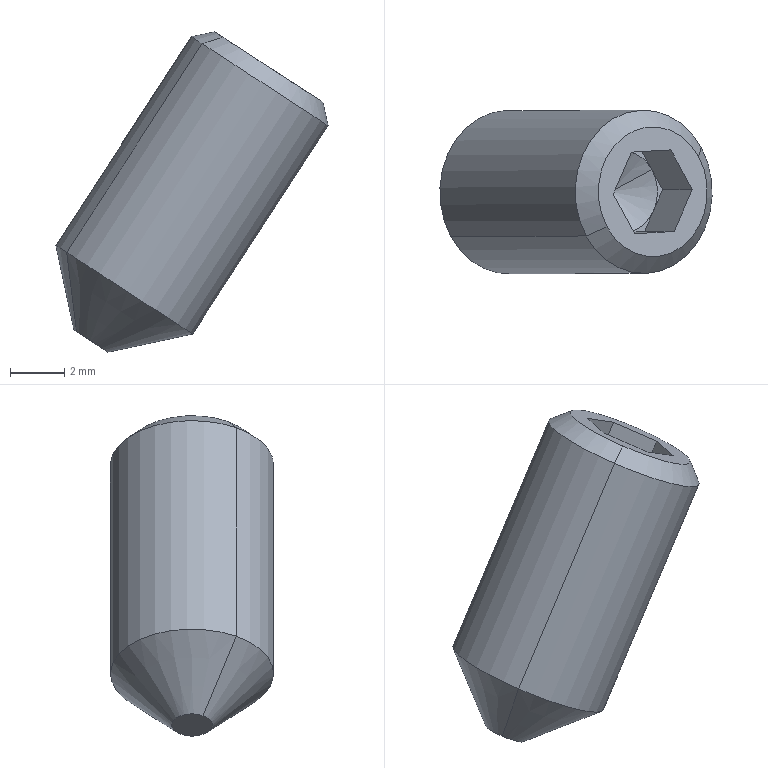Component | SolidWorks | SetScrewTAY12-M6-L12(YIHEDA)-1 | 1 solid | 22 faces | box 10.01 x 6 x 11.77 mm | volume 283 mm3 | plane 14 | cone 6 | cylinder 2 | commonest cylinder face diameters 6 x2
STEP:
#1=CARTESIAN_POINT('',(4.498,-0.6106,10.849));
#2=VERTEX_POINT('',#1);
#3=CARTESIAN_POINT('',(4.332,-0.7385,10.958));
#4=VERTEX_POINT('',#3);
#5=CARTESIAN_POINT('',(4.415,-0.6746,10.903));
#6=DIRECTION('',(-0.5446,0.,-0.8387));
#7=DIRECTION('',(-0.705,-0.5417,0.4578));
#8=AXIS2_PLACEMENT_3D('',#5,#6,#7);
#9=CIRCLE('',#8,0.1181);
#10=EDGE_CURVE('',#2,#4,#9,.T.);
#11=ORIENTED_EDGE('',*,*,#10,.F.);
#12=CARTESIAN_POINT('',(4.694,-0.6106,11.151));
#13=VERTEX_POINT('',#12);
#14=CARTESIAN_POINT('',(4.45,-0.6106,10.775));
#15=DIRECTION('',(0.5446,-0.,0.8387));
#16=VECTOR('',#15,39.37);
#17=LINE('',#14,#16);
#18=EDGE_CURVE('',#2,#13,#17,.T.);
#19=ORIENTED_EDGE('',*,*,#18,.T.);
#20=CARTESIAN_POINT('',(4.528,-0.7385,11.259));
#21=VERTEX_POINT('',#20);
#22=CARTESIAN_POINT('',(4.611,-0.6746,11.205));
#23=DIRECTION('',(-0.5446,0.,-0.8387));
#24=DIRECTION('',(-0.705,-0.5417,0.4578));
#25=AXIS2_PLACEMENT_3D('',#22,#23,#24);
#26=CIRCLE('',#25,0.1181);
#27=EDGE_CURVE('',#13,#21,#26,.T.);
#28=ORIENTED_EDGE('',*,*,#27,.T.);
#29=CARTESIAN_POINT('',(4.284,-0.7385,10.883));
#30=DIRECTION('',(0.5446,-0.,0.8387));
#31=VECTOR('',#30,39.37);
#32=LINE('',#29,#31);
#33=EDGE_CURVE('',#4,#21,#32,.T.);
#34=ORIENTED_EDGE('',*,*,#33,.F.);
#35=EDGE_LOOP('',(#11,#19,#28,#34));
#36=FACE_OUTER_BOUND('',#35,.T.);
#37=CARTESIAN_POINT('',(4.367,-0.6746,10.829));
#38=DIRECTION('',(0.5446,-0.,0.8387));
#39=DIRECTION('',(-0.705,-0.5417,0.4578));
#40=AXIS2_PLACEMENT_3D('',#37,#38,#39);
#41=CYLINDRICAL_SURFACE('',#40,0.1181);
#42=ADVANCED_FACE('',(#36),#41,.T.);
#43=CARTESIAN_POINT('',(4.346,-0.6906,10.843));
#44=VERTEX_POINT('',#43);
#45=CARTESIAN_POINT('',(4.388,-0.6586,10.816));
#46=VERTEX_POINT('',#45);
#47=CARTESIAN_POINT('',(4.367,-0.6746,10.829));
#48=DIRECTION('',(-0.5446,0.,-0.8387));
#49=DIRECTION('',(-0.705,-0.5417,0.4578));
#50=AXIS2_PLACEMENT_3D('',#47,#48,#49);
#51=CIRCLE('',#50,0.02953);
#52=EDGE_CURVE('',#44,#46,#51,.T.);
#53=ORIENTED_EDGE('',*,*,#52,.F.);
#54=CARTESIAN_POINT('',(4.332,-0.7385,10.958));
#55=DIRECTION('',(-0.1134,-0.3831,0.9167));
#56=VECTOR('',#55,39.37);
#57=LINE('',#54,#56);
#58=EDGE_CURVE('',#44,#4,#57,.T.);
#59=ORIENTED_EDGE('',*,*,#58,.T.);
#60=CARTESIAN_POINT('',(4.415,-0.6746,10.903));
#61=DIRECTION('',(-0.5446,0.,-0.8387));
#62=DIRECTION('',(-0.705,-0.5417,0.4578));
#63=AXIS2_PLACEMENT_3D('',#60,#61,#62);
#64=CIRCLE('',#63,0.1181);
#65=EDGE_CURVE('',#4,#2,#64,.T.);
#66=ORIENTED_EDGE('',*,*,#65,.T.);
#67=CARTESIAN_POINT('',(4.498,-0.6106,10.849));
#68=DIRECTION('',(0.8836,0.3831,0.2693));
#69=VECTOR('',#68,39.37);
#70=LINE('',#67,#69);
#71=EDGE_CURVE('',#46,#2,#70,.T.);
#72=ORIENTED_EDGE('',*,*,#71,.F.);
#73=EDGE_LOOP('',(#53,#59,#66,#72));
#74=FACE_OUTER_BOUND('',#73,.T.);
#75=CARTESIAN_POINT('',(4.415,-0.6746,10.903));
#76=DIRECTION('',(0.5446,-0.,0.8387));
#77=DIRECTION('',(0.705,0.5417,-0.4578));
#78=AXIS2_PLACEMENT_3D('',#75,#76,#77);
#79=CONICAL_SURFACE('',#78,0.1181,0.7854);
#80=ADVANCED_FACE('',(#74),#79,.T.);
#81=CARTESIAN_POINT('',(4.558,-0.7255,11.268));
#82=VERTEX_POINT('',#81);
#83=CARTESIAN_POINT('',(4.691,-0.6237,11.182));
#84=VERTEX_POINT('',#83);
#85=CARTESIAN_POINT('',(4.624,-0.6746,11.225));
#86=DIRECTION('',(-0.5446,0.,-0.8387));
#87=DIRECTION('',(-0.705,-0.5417,0.4578));
#88=AXIS2_PLACEMENT_3D('',#85,#86,#87);
#89=CIRCLE('',#88,0.09396);
#90=EDGE_CURVE('',#82,#84,#89,.T.);
#91=ORIENTED_EDGE('',*,*,#90,.T.);
#92=CARTESIAN_POINT('',(4.691,-0.6237,11.182));
#93=DIRECTION('',(0.1134,0.3831,-0.9167));
#94=VECTOR('',#93,39.37);
#95=LINE('',#92,#94);
#96=EDGE_CURVE('',#84,#13,#95,.T.);
#97=ORIENTED_EDGE('',*,*,#96,.T.);
#98=CARTESIAN_POINT('',(4.611,-0.6746,11.205));
#99=DIRECTION('',(-0.5446,0.,-0.8387));
#100=DIRECTION('',(-0.705,-0.5417,0.4578));
#101=AXIS2_PLACEMENT_3D('',#98,#99,#100);
#102=CIRCLE('',#101,0.1181);
#103=EDGE_CURVE('',#21,#13,#102,.T.);
#104=ORIENTED_EDGE('',*,*,#103,.F.);
#105=CARTESIAN_POINT('',(4.558,-0.7255,11.268));
#106=DIRECTION('',(-0.8836,-0.3831,-0.2693));
#107=VECTOR('',#106,39.37);
#108=LINE('',#105,#107);
#109=EDGE_CURVE('',#82,#21,#108,.T.);
#110=ORIENTED_EDGE('',*,*,#109,.F.);
#111=EDGE_LOOP('',(#91,#97,#104,#110));
#112=FACE_OUTER_BOUND('',#111,.T.);
#113=CARTESIAN_POINT('',(4.624,-0.6746,11.225));
#114=DIRECTION('',(-0.5446,0.,-0.8387));
#115=DIRECTION('',(-0.705,-0.5417,0.4578));
#116=AXIS2_PLACEMENT_3D('',#113,#114,#115);
#117=CONICAL_SURFACE('',#116,0.09396,0.7854);
#118=ADVANCED_FACE('',(#112),#117,.T.);
#119=CARTESIAN_POINT('',(4.563,-0.6746,11.131));
#120=VERTEX_POINT('',#119);
#121=CARTESIAN_POINT('',(4.623,-0.6426,11.132));
#122=VERTEX_POINT('',#121);
#123=CARTESIAN_POINT('',(4.623,-0.6426,11.132));
#124=DIRECTION('',(0.8818,0.4713,0.01518));
#125=VECTOR('',#124,39.37);
#126=LINE('',#123,#125);
#127=EDGE_CURVE('',#120,#122,#126,.T.);
#128=ORIENTED_EDGE('',*,*,#127,.F.);
#129=CARTESIAN_POINT('',(4.54,-0.7066,11.186));
#130=VERTEX_POINT('',#129);
#131=CARTESIAN_POINT('',(4.54,-0.7066,11.186));
#132=DIRECTION('',(-0.3448,-0.4713,0.8118));
#133=VECTOR('',#132,39.37);
#134=LINE('',#131,#133);
#135=EDGE_CURVE('',#120,#130,#134,.T.);
#136=ORIENTED_EDGE('',*,*,#135,.T.);
#137=CARTESIAN_POINT('',(4.584,-0.7336,11.158));
#138=VERTEX_POINT('',#137);
#139=CARTESIAN_POINT('',(4.581,-0.6746,11.159));
#140=DIRECTION('',(0.5446,-0.,0.8387));
#141=DIRECTION('',(-0.705,-0.5417,0.4578));
#142=AXIS2_PLACEMENT_3D('',#139,#140,#141);
#143=CIRCLE('',#142,0.05906);
#144=EDGE_CURVE('',#130,#138,#143,.T.);
#145=ORIENTED_EDGE('',*,*,#144,.T.);
#146=CARTESIAN_POINT('',(4.625,-0.7016,11.131));
#147=VERTEX_POINT('',#146);
#148=CARTESIAN_POINT('',(4.581,-0.6746,11.159));
#149=DIRECTION('',(0.5446,-0.,0.8387));
#150=DIRECTION('',(-0.705,-0.5417,0.4578));
#151=AXIS2_PLACEMENT_3D('',#148,#149,#150);
#152=CIRCLE('',#151,0.05906);
#153=EDGE_CURVE('',#138,#147,#152,.T.);
#154=ORIENTED_EDGE('',*,*,#153,.T.);
#155=CARTESIAN_POINT('',(4.581,-0.6746,11.159));
#156=DIRECTION('',(0.5446,-0.,0.8387));
#157=DIRECTION('',(-0.705,-0.5417,0.4578));
#158=AXIS2_PLACEMENT_3D('',#155,#156,#157);
#159=CIRCLE('',#158,0.05906);
#160=EDGE_CURVE('',#147,#122,#159,.T.);
#161=ORIENTED_EDGE('',*,*,#160,.T.);
#162=EDGE_LOOP('',(#128,#136,#145,#154,#161));
#163=FACE_OUTER_BOUND('',#162,.T.);
#164=CARTESIAN_POINT('',(4.581,-0.6746,11.159));
#165=DIRECTION('',(0.5446,-0.,0.8387));
#166=DIRECTION('',(0.705,0.5417,-0.4578));
#167=AXIS2_PLACEMENT_3D('',#164,#165,#166);
#168=CONICAL_SURFACE('',#167,0.05906,1.055);
#169=ADVANCED_FACE('',(#163),#168,.F.);
#170=ORIENTED_EDGE('',*,*,#153,.F.);
#171=CARTESIAN_POINT('',(4.612,-0.7319,11.139));
#172=VERTEX_POINT('',#171);
#173=CARTESIAN_POINT('',(4.612,-0.7319,11.139));
#174=DIRECTION('',(-0.8377,-0.04887,0.544));
#175=VECTOR('',#174,39.37);
#176=LINE('',#173,#175);
#177=EDGE_CURVE('',#172,#138,#176,.T.);
#178=ORIENTED_EDGE('',*,*,#177,.F.);
#179=CARTESIAN_POINT('',(4.639,-0.6712,11.122));
#180=DIRECTION('',(-0.3833,-0.8894,0.2489));
#181=VECTOR('',#180,39.37);
#182=LINE('',#179,#181);
#183=EDGE_CURVE('',#147,#172,#182,.T.);
#184=ORIENTED_EDGE('',*,*,#183,.F.);
#185=EDGE_LOOP('',(#170,#178,#184));
#186=FACE_OUTER_BOUND('',#185,.T.);
#187=CARTESIAN_POINT('',(4.581,-0.6746,11.159));
#188=DIRECTION('',(-0.5446,0.,-0.8387));
#189=DIRECTION('',(-0.4543,0.8406,0.295));
#190=AXIS2_PLACEMENT_3D('',#187,#188,#189);
#191=PLANE('',#190);
#192=ADVANCED_FACE('',(#186),#191,.F.);
#193=ORIENTED_EDGE('',*,*,#90,.F.);
#194=CARTESIAN_POINT('',(4.624,-0.6746,11.225));
#195=DIRECTION('',(-0.5446,0.,-0.8387));
#196=DIRECTION('',(-0.705,-0.5417,0.4578));
#197=AXIS2_PLACEMENT_3D('',#194,#195,#196);
#198=CIRCLE('',#197,0.09396);
#199=EDGE_CURVE('',#84,#82,#198,.T.);
#200=ORIENTED_EDGE('',*,*,#199,.F.);
#201=EDGE_LOOP('',(#193,#200));
#202=FACE_OUTER_BOUND('',#201,.T.);
#203=CARTESIAN_POINT('',(4.593,-0.6172,11.246));
#204=VERTEX_POINT('',#203);
#205=CARTESIAN_POINT('',(4.65,-0.6139,11.208));
#206=VERTEX_POINT('',#205);
#207=CARTESIAN_POINT('',(4.593,-0.6172,11.246));
#208=DIRECTION('',(0.8377,0.04887,-0.544));
#209=VECTOR('',#208,39.37);
#210=LINE('',#207,#209);
#211=EDGE_CURVE('',#204,#206,#210,.T.);
#212=ORIENTED_EDGE('',*,*,#211,.T.);
#213=CARTESIAN_POINT('',(4.681,-0.6712,11.188));
#214=VERTEX_POINT('',#213);
#215=CARTESIAN_POINT('',(4.65,-0.6139,11.208));
#216=DIRECTION('',(0.4543,-0.8406,-0.295));
#217=VECTOR('',#216,39.37);
#218=LINE('',#215,#217);
#219=EDGE_CURVE('',#206,#214,#218,.T.);
#220=ORIENTED_EDGE('',*,*,#219,.T.);
#221=CARTESIAN_POINT('',(4.655,-0.7319,11.205));
#222=VERTEX_POINT('',#221);
#223=CARTESIAN_POINT('',(4.681,-0.6712,11.188));
#224=DIRECTION('',(-0.3833,-0.8894,0.2489));
#225=VECTOR('',#224,39.37);
#226=LINE('',#223,#225);
#227=EDGE_CURVE('',#214,#222,#226,.T.);
#228=ORIENTED_EDGE('',*,*,#227,.T.);
#229=CARTESIAN_POINT('',(4.598,-0.7352,11.242));
#230=VERTEX_POINT('',#229);
#231=CARTESIAN_POINT('',(4.655,-0.7319,11.205));
#232=DIRECTION('',(-0.8377,-0.04887,0.544));
#233=VECTOR('',#232,39.37);
#234=LINE('',#231,#233);
#235=EDGE_CURVE('',#222,#230,#234,.T.);
#236=ORIENTED_EDGE('',*,*,#235,.T.);
#237=CARTESIAN_POINT('',(4.567,-0.6779,11.262));
#238=VERTEX_POINT('',#237);
#239=CARTESIAN_POINT('',(4.598,-0.7352,11.242));
#240=DIRECTION('',(-0.4543,0.8406,0.295));
#241=VECTOR('',#240,39.37);
#242=LINE('',#239,#241);
#243=EDGE_CURVE('',#230,#238,#242,.T.);
#244=ORIENTED_EDGE('',*,*,#243,.T.);
#245=CARTESIAN_POINT('',(4.567,-0.6779,11.262));
#246=DIRECTION('',(0.3833,0.8894,-0.2489));
#247=VECTOR('',#246,39.37);
#248=LINE('',#245,#247);
#249=EDGE_CURVE('',#238,#204,#248,.T.);
#250=ORIENTED_EDGE('',*,*,#249,.T.);
#251=EDGE_LOOP('',(#212,#220,#228,#236,#244,#250));
#252=FACE_BOUND('',#251,.T.);
#253=CARTESIAN_POINT('',(4.624,-0.6746,11.225));
#254=DIRECTION('',(-0.5446,0.,-0.8387));
#255=DIRECTION('',(-0.4543,0.8406,0.295));
#256=AXIS2_PLACEMENT_3D('',#253,#254,#255);
#257=PLANE('',#256);
#258=ADVANCED_FACE('',(#202,#252),#257,.F.);
#259=ORIENTED_EDGE('',*,*,#135,.F.);
#260=ORIENTED_EDGE('',*,*,#127,.T.);
#261=CARTESIAN_POINT('',(4.579,-0.6156,11.161));
#262=VERTEX_POINT('',#261);
#263=CARTESIAN_POINT('',(4.581,-0.6746,11.159));
#264=DIRECTION('',(0.5446,-0.,0.8387));
#265=DIRECTION('',(-0.705,-0.5417,0.4578));
#266=AXIS2_PLACEMENT_3D('',#263,#264,#265);
#267=CIRCLE('',#266,0.05906);
#268=EDGE_CURVE('',#122,#262,#267,.T.);
#269=ORIENTED_EDGE('',*,*,#268,.T.);
#270=CARTESIAN_POINT('',(4.537,-0.6476,11.188));
#271=VERTEX_POINT('',#270);
#272=CARTESIAN_POINT('',(4.581,-0.6746,11.159));
#273=DIRECTION('',(0.5446,-0.,0.8387));
#274=DIRECTION('',(-0.705,-0.5417,0.4578));
#275=AXIS2_PLACEMENT_3D('',#272,#273,#274);
#276=CIRCLE('',#275,0.05906);
#277=EDGE_CURVE('',#262,#271,#276,.T.);
#278=ORIENTED_EDGE('',*,*,#277,.T.);
#279=CARTESIAN_POINT('',(4.581,-0.6746,11.159));
#280=DIRECTION('',(0.5446,-0.,0.8387));
#281=DIRECTION('',(-0.705,-0.5417,0.4578));
#282=AXIS2_PLACEMENT_3D('',#279,#280,#281);
#283=CIRCLE('',#282,0.05906);
#284=EDGE_CURVE('',#271,#130,#283,.T.);
#285=ORIENTED_EDGE('',*,*,#284,.T.);
#286=EDGE_LOOP('',(#259,#260,#269,#278,#285));
#287=FACE_OUTER_BOUND('',#286,.T.);
#288=CARTESIAN_POINT('',(4.581,-0.6746,11.159));
#289=DIRECTION('',(0.5446,-0.,0.8387));
#290=DIRECTION('',(0.705,0.5417,-0.4578));
#291=AXIS2_PLACEMENT_3D('',#288,#289,#290);
#292=CONICAL_SURFACE('',#291,0.05906,1.055);
#293=ADVANCED_FACE('',(#287),#292,.F.);
#294=ORIENTED_EDGE('',*,*,#249,.F.);
#295=CARTESIAN_POINT('',(4.524,-0.6779,11.196));
#296=VERTEX_POINT('',#295);
#297=CARTESIAN_POINT('',(4.524,-0.6779,11.196));
#298=DIRECTION('',(0.5446,-0.,0.8387));
#299=VECTOR('',#298,39.37);
#300=LINE('',#297,#299);
#301=EDGE_CURVE('',#296,#238,#300,.T.);
#302=ORIENTED_EDGE('',*,*,#301,.F.);
#303=CARTESIAN_POINT('',(4.524,-0.6779,11.196));
#304=DIRECTION('',(0.3833,0.8894,-0.2489));
#305=VECTOR('',#304,39.37);
#306=LINE('',#303,#305);
#307=EDGE_CURVE('',#296,#271,#306,.T.);
#308=ORIENTED_EDGE('',*,*,#307,.T.);
#309=CARTESIAN_POINT('',(4.55,-0.6172,11.179));
#310=VERTEX_POINT('',#309);
#311=CARTESIAN_POINT('',(4.524,-0.6779,11.196));
#312=DIRECTION('',(0.3833,0.8894,-0.2489));
#313=VECTOR('',#312,39.37);
#314=LINE('',#311,#313);
#315=EDGE_CURVE('',#271,#310,#314,.T.);
#316=ORIENTED_EDGE('',*,*,#315,.T.);
#317=CARTESIAN_POINT('',(4.55,-0.6172,11.179));
#318=DIRECTION('',(0.5446,-0.,0.8387));
#319=VECTOR('',#318,39.37);
#320=LINE('',#317,#319);
#321=EDGE_CURVE('',#310,#204,#320,.T.);
#322=ORIENTED_EDGE('',*,*,#321,.T.);
#323=EDGE_LOOP('',(#294,#302,#308,#316,#322));
#324=FACE_OUTER_BOUND('',#323,.T.);
#325=CARTESIAN_POINT('',(4.524,-0.6779,11.196));
#326=DIRECTION('',(0.7459,-0.4571,-0.4844));
#327=DIRECTION('',(0.5446,-0.,0.8387));
#328=AXIS2_PLACEMENT_3D('',#325,#326,#327);
#329=PLANE('',#328);
#330=ADVANCED_FACE('',(#324),#329,.T.);
#331=ORIENTED_EDGE('',*,*,#268,.F.);
#332=CARTESIAN_POINT('',(4.608,-0.6139,11.142));
#333=VERTEX_POINT('',#332);
#334=CARTESIAN_POINT('',(4.608,-0.6139,11.142));
#335=DIRECTION('',(0.4543,-0.8406,-0.295));
#336=VECTOR('',#335,39.37);
#337=LINE('',#334,#336);
#338=EDGE_CURVE('',#333,#122,#337,.T.);
#339=ORIENTED_EDGE('',*,*,#338,.F.);
#340=CARTESIAN_POINT('',(4.55,-0.6172,11.179));
#341=DIRECTION('',(0.8377,0.04887,-0.544));
#342=VECTOR('',#341,39.37);
#343=LINE('',#340,#342);
#344=EDGE_CURVE('',#262,#333,#343,.T.);
#345=ORIENTED_EDGE('',*,*,#344,.F.);
#346=EDGE_LOOP('',(#331,#339,#345));
#347=FACE_OUTER_BOUND('',#346,.T.);
#348=CARTESIAN_POINT('',(4.581,-0.6746,11.159));
#349=DIRECTION('',(-0.5446,0.,-0.8387));
#350=DIRECTION('',(-0.4543,0.8406,0.295));
#351=AXIS2_PLACEMENT_3D('',#348,#349,#350);
#352=PLANE('',#351);
#353=ADVANCED_FACE('',(#347),#352,.F.);
#354=ORIENTED_EDGE('',*,*,#211,.F.);
#355=ORIENTED_EDGE('',*,*,#321,.F.);
#356=CARTESIAN_POINT('',(4.55,-0.6172,11.179));
#357=DIRECTION('',(0.8377,0.04887,-0.544));
#358=VECTOR('',#357,39.37);
#359=LINE('',#356,#358);
#360=EDGE_CURVE('',#310,#262,#359,.T.);
#361=ORIENTED_EDGE('',*,*,#360,.T.);
#362=ORIENTED_EDGE('',*,*,#344,.T.);
#363=CARTESIAN_POINT('',(4.608,-0.6139,11.142));
#364=DIRECTION('',(0.5446,-0.,0.8387));
#365=VECTOR('',#364,39.37);
#366=LINE('',#363,#365);
#367=EDGE_CURVE('',#333,#206,#366,.T.);
#368=ORIENTED_EDGE('',*,*,#367,.T.);
#369=EDGE_LOOP('',(#354,#355,#361,#362,#368));
#370=FACE_OUTER_BOUND('',#369,.T.);
#371=CARTESIAN_POINT('',(4.55,-0.6172,11.179));
#372=DIRECTION('',(0.04098,-0.9988,-0.02661));
#373=DIRECTION('',(-0.8377,-0.04887,0.544));
#374=AXIS2_PLACEMENT_3D('',#371,#372,#373);
#375=PLANE('',#374);
#376=ADVANCED_FACE('',(#370),#375,.T.);
#377=ORIENTED_EDGE('',*,*,#144,.F.);
#378=CARTESIAN_POINT('',(4.555,-0.7352,11.176));
#379=VERTEX_POINT('',#378);
#380=CARTESIAN_POINT('',(4.555,-0.7352,11.176));
#381=DIRECTION('',(-0.4543,0.8406,0.295));
#382=VECTOR('',#381,39.37);
#383=LINE('',#380,#382);
#384=EDGE_CURVE('',#379,#130,#383,.T.);
#385=ORIENTED_EDGE('',*,*,#384,.F.);
#386=CARTESIAN_POINT('',(4.612,-0.7319,11.139));
#387=DIRECTION('',(-0.8377,-0.04887,0.544));
#388=VECTOR('',#387,39.37);
#389=LINE('',#386,#388);
#390=EDGE_CURVE('',#138,#379,#389,.T.);
#391=ORIENTED_EDGE('',*,*,#390,.F.);
#392=EDGE_LOOP('',(#377,#385,#391));
#393=FACE_OUTER_BOUND('',#392,.T.);
#394=CARTESIAN_POINT('',(4.581,-0.6746,11.159));
#395=DIRECTION('',(-0.5446,0.,-0.8387));
#396=DIRECTION('',(-0.4543,0.8406,0.295));
#397=AXIS2_PLACEMENT_3D('',#394,#395,#396);
#398=PLANE('',#397);
#399=ADVANCED_FACE('',(#393),#398,.F.);
#400=ORIENTED_EDGE('',*,*,#235,.F.);
#401=CARTESIAN_POINT('',(4.612,-0.7319,11.139));
#402=DIRECTION('',(0.5446,-0.,0.8387));
#403=VECTOR('',#402,39.37);
#404=LINE('',#401,#403);
#405=EDGE_CURVE('',#172,#222,#404,.T.);
#406=ORIENTED_EDGE('',*,*,#405,.F.);
#407=ORIENTED_EDGE('',*,*,#177,.T.);
#408=ORIENTED_EDGE('',*,*,#390,.T.);
#409=CARTESIAN_POINT('',(4.555,-0.7352,11.176));
#410=DIRECTION('',(0.5446,-0.,0.8387));
#411=VECTOR('',#410,39.37);
#412=LINE('',#409,#411);
#413=EDGE_CURVE('',#379,#230,#412,.T.);
#414=ORIENTED_EDGE('',*,*,#413,.T.);
#415=EDGE_LOOP('',(#400,#406,#407,#408,#414));
#416=FACE_OUTER_BOUND('',#415,.T.);
#417=CARTESIAN_POINT('',(4.612,-0.7319,11.139));
#418=DIRECTION('',(-0.04098,0.9988,0.02661));
#419=DIRECTION('',(-0.5446,0.,-0.8387));
#420=AXIS2_PLACEMENT_3D('',#417,#418,#419);
#421=PLANE('',#420);
#422=ADVANCED_FACE('',(#416),#421,.T.);
#423=ORIENTED_EDGE('',*,*,#227,.F.);
#424=CARTESIAN_POINT('',(4.639,-0.6712,11.122));
#425=VERTEX_POINT('',#424);
#426=CARTESIAN_POINT('',(4.639,-0.6712,11.122));
#427=DIRECTION('',(0.5446,-0.,0.8387));
#428=VECTOR('',#427,39.37);
#429=LINE('',#426,#428);
#430=EDGE_CURVE('',#425,#214,#429,.T.);
#431=ORIENTED_EDGE('',*,*,#430,.F.);
#432=CARTESIAN_POINT('',(4.639,-0.6712,11.122));
#433=DIRECTION('',(-0.3833,-0.8894,0.2489));
#434=VECTOR('',#433,39.37);
#435=LINE('',#432,#434);
#436=EDGE_CURVE('',#425,#147,#435,.T.);
#437=ORIENTED_EDGE('',*,*,#436,.T.);
#438=ORIENTED_EDGE('',*,*,#183,.T.);
#439=ORIENTED_EDGE('',*,*,#405,.T.);
#440=EDGE_LOOP('',(#423,#431,#437,#438,#439));
#441=FACE_OUTER_BOUND('',#440,.T.);
#442=CARTESIAN_POINT('',(4.639,-0.6712,11.122));
#443=DIRECTION('',(-0.7459,0.4571,0.4844));
#444=DIRECTION('',(0.5446,-0.,0.8387));
#445=AXIS2_PLACEMENT_3D('',#442,#443,#444);
#446=PLANE('',#445);
#447=ADVANCED_FACE('',(#441),#446,.T.);
#448=ORIENTED_EDGE('',*,*,#160,.F.);
#449=ORIENTED_EDGE('',*,*,#436,.F.);
#450=CARTESIAN_POINT('',(4.608,-0.6139,11.142));
#451=DIRECTION('',(0.4543,-0.8406,-0.295));
#452=VECTOR('',#451,39.37);
#453=LINE('',#450,#452);
#454=EDGE_CURVE('',#122,#425,#453,.T.);
#455=ORIENTED_EDGE('',*,*,#454,.F.);
#456=EDGE_LOOP('',(#448,#449,#455));
#457=FACE_OUTER_BOUND('',#456,.T.);
#458=CARTESIAN_POINT('',(4.581,-0.6746,11.159));
#459=DIRECTION('',(-0.5446,0.,-0.8387));
#460=DIRECTION('',(-0.4543,0.8406,0.295));
#461=AXIS2_PLACEMENT_3D('',#458,#459,#460);
#462=PLANE('',#461);
#463=ADVANCED_FACE('',(#457),#462,.F.);
#464=ORIENTED_EDGE('',*,*,#219,.F.);
#465=ORIENTED_EDGE('',*,*,#367,.F.);
#466=ORIENTED_EDGE('',*,*,#338,.T.);
#467=ORIENTED_EDGE('',*,*,#454,.T.);
#468=ORIENTED_EDGE('',*,*,#430,.T.);
#469=EDGE_LOOP('',(#464,#465,#466,#467,#468));
#470=FACE_OUTER_BOUND('',#469,.T.);
#471=CARTESIAN_POINT('',(4.608,-0.6139,11.142));
#472=DIRECTION('',(-0.705,-0.5417,0.4578));
#473=DIRECTION('',(0.4543,-0.8406,-0.295));
#474=AXIS2_PLACEMENT_3D('',#471,#472,#473);
#475=PLANE('',#474);
#476=ADVANCED_FACE('',(#470),#475,.T.);
#477=ORIENTED_EDGE('',*,*,#277,.F.);
#478=ORIENTED_EDGE('',*,*,#360,.F.);
#479=ORIENTED_EDGE('',*,*,#315,.F.);
#480=EDGE_LOOP('',(#477,#478,#479));
#481=FACE_OUTER_BOUND('',#480,.T.);
#482=CARTESIAN_POINT('',(4.581,-0.6746,11.159));
#483=DIRECTION('',(-0.5446,0.,-0.8387));
#484=DIRECTION('',(-0.4543,0.8406,0.295));
#485=AXIS2_PLACEMENT_3D('',#482,#483,#484);
#486=PLANE('',#485);
#487=ADVANCED_FACE('',(#481),#486,.F.);
#488=ORIENTED_EDGE('',*,*,#284,.F.);
#489=ORIENTED_EDGE('',*,*,#307,.F.);
#490=CARTESIAN_POINT('',(4.555,-0.7352,11.176));
#491=DIRECTION('',(-0.4543,0.8406,0.295));
#492=VECTOR('',#491,39.37);
#493=LINE('',#490,#492);
#494=EDGE_CURVE('',#130,#296,#493,.T.);
#495=ORIENTED_EDGE('',*,*,#494,.F.);
#496=EDGE_LOOP('',(#488,#489,#495));
#497=FACE_OUTER_BOUND('',#496,.T.);
#498=CARTESIAN_POINT('',(4.581,-0.6746,11.159));
#499=DIRECTION('',(-0.5446,0.,-0.8387));
#500=DIRECTION('',(-0.4543,0.8406,0.295));
#501=AXIS2_PLACEMENT_3D('',#498,#499,#500);
#502=PLANE('',#501);
#503=ADVANCED_FACE('',(#497),#502,.F.);
#504=ORIENTED_EDGE('',*,*,#96,.F.);
#505=ORIENTED_EDGE('',*,*,#199,.T.);
#506=ORIENTED_EDGE('',*,*,#109,.T.);
#507=ORIENTED_EDGE('',*,*,#27,.F.);
#508=EDGE_LOOP('',(#504,#505,#506,#507));
#509=FACE_OUTER_BOUND('',#508,.T.);
#510=CARTESIAN_POINT('',(4.624,-0.6746,11.225));
#511=DIRECTION('',(-0.5446,0.,-0.8387));
#512=DIRECTION('',(-0.705,-0.5417,0.4578));
#513=AXIS2_PLACEMENT_3D('',#510,#511,#512);
#514=CONICAL_SURFACE('',#513,0.09396,0.7854);
#515=ADVANCED_FACE('',(#509),#514,.T.);
#516=ORIENTED_EDGE('',*,*,#243,.F.);
#517=ORIENTED_EDGE('',*,*,#413,.F.);
#518=ORIENTED_EDGE('',*,*,#384,.T.);
#519=ORIENTED_EDGE('',*,*,#494,.T.);
#520=ORIENTED_EDGE('',*,*,#301,.T.);
#521=EDGE_LOOP('',(#516,#517,#518,#519,#520));
#522=FACE_OUTER_BOUND('',#521,.T.);
#523=CARTESIAN_POINT('',(4.555,-0.7352,11.176));
#524=DIRECTION('',(0.705,0.5417,-0.4578));
#525=DIRECTION('',(-0.5446,0.,-0.8387));
#526=AXIS2_PLACEMENT_3D('',#523,#524,#525);
#527=PLANE('',#526);
#528=ADVANCED_FACE('',(#522),#527,.T.);
#529=CARTESIAN_POINT('',(4.367,-0.6746,10.829));
#530=DIRECTION('',(-0.5446,0.,-0.8387));
#531=DIRECTION('',(-0.705,-0.5417,0.4578));
#532=AXIS2_PLACEMENT_3D('',#529,#530,#531);
#533=CIRCLE('',#532,0.02953);
#534=EDGE_CURVE('',#46,#44,#533,.T.);
#535=ORIENTED_EDGE('',*,*,#534,.T.);
#536=ORIENTED_EDGE('',*,*,#52,.T.);
#537=EDGE_LOOP('',(#535,#536));
#538=FACE_OUTER_BOUND('',#537,.T.);
#539=CARTESIAN_POINT('',(4.354,-0.6497,10.838));
#540=DIRECTION('',(0.5446,-0.,0.8387));
#541=DIRECTION('',(0.705,0.5417,-0.4578));
#542=AXIS2_PLACEMENT_3D('',#539,#540,#541);
#543=PLANE('',#542);
#544=ADVANCED_FACE('',(#538),#543,.F.);
#545=ORIENTED_EDGE('',*,*,#58,.F.);
#546=ORIENTED_EDGE('',*,*,#534,.F.);
#547=ORIENTED_EDGE('',*,*,#71,.T.);
#548=ORIENTED_EDGE('',*,*,#10,.T.);
#549=EDGE_LOOP('',(#545,#546,#547,#548));
#550=FACE_OUTER_BOUND('',#549,.T.);
#551=CARTESIAN_POINT('',(4.415,-0.6746,10.903));
#552=DIRECTION('',(0.5446,-0.,0.8387));
#553=DIRECTION('',(0.705,0.5417,-0.4578));
#554=AXIS2_PLACEMENT_3D('',#551,#552,#553);
#555=CONICAL_SURFACE('',#554,0.1181,0.7854);
#556=ADVANCED_FACE('',(#550),#555,.T.);
#557=ORIENTED_EDGE('',*,*,#18,.F.);
#558=ORIENTED_EDGE('',*,*,#65,.F.);
#559=ORIENTED_EDGE('',*,*,#33,.T.);
#560=ORIENTED_EDGE('',*,*,#103,.T.);
#561=EDGE_LOOP('',(#557,#558,#559,#560));
#562=FACE_OUTER_BOUND('',#561,.T.);
#563=CARTESIAN_POINT('',(4.367,-0.6746,10.829));
#564=DIRECTION('',(0.5446,-0.,0.8387));
#565=DIRECTION('',(-0.705,-0.5417,0.4578));
#566=AXIS2_PLACEMENT_3D('',#563,#564,#565);
#567=CYLINDRICAL_SURFACE('',#566,0.1181);
#568=ADVANCED_FACE('',(#562),#567,.T.);
#569=CLOSED_SHELL('',(#42,#80,#118,#169,#192,#258,#293,#330,#353,#376,#399,#422,#447,#463,#476,#487,#503,#515,#528,#544,#556,#568));
#570=MANIFOLD_SOLID_BREP('',#569);
#571=CARTESIAN_POINT('',(0.,0.,0.));
#572=DIRECTION('',(0.,0.,1.));
#573=DIRECTION('',(1.,0.,0.));
#574=AXIS2_PLACEMENT_3D('',#571,#572,#573);
#575=(LENGTH_UNIT()NAMED_UNIT(*)SI_UNIT($,.METRE.));
#576=LENGTH_MEASURE_WITH_UNIT(LENGTH_MEASURE(0.0254),#575);
#577=DIMENSIONAL_EXPONENTS(1.,0.,0.,0.,0.,0.,0.);
#578=(CONVERSION_BASED_UNIT('',#576)LENGTH_UNIT()NAMED_UNIT(#577));
#579=UNCERTAINTY_MEASURE_WITH_UNIT(LENGTH_MEASURE(0.00001),#578,'','');
#580=(NAMED_UNIT(*)PLANE_ANGLE_UNIT()SI_UNIT($,.RADIAN.));
#581=(NAMED_UNIT(*)SI_UNIT($,.STERADIAN.)SOLID_ANGLE_UNIT());
#582=(GEOMETRIC_REPRESENTATION_CONTEXT(3)GLOBAL_UNCERTAINTY_ASSIGNED_CONTEXT((#579))GLOBAL_UNIT_ASSIGNED_CONTEXT((#578,#580,#581))REPRESENTATION_CONTEXT('',''));
#583=ADVANCED_BREP_SHAPE_REPRESENTATION('',(#570,#574),#582);
#584=COLOUR_RGB('',0.7922,0.8196,0.9333);
#585=FILL_AREA_STYLE_COLOUR('',#584);
#586=FILL_AREA_STYLE('',(#585));
#587=SURFACE_STYLE_FILL_AREA(#586);
#588=SURFACE_SIDE_STYLE('',(#587));
#589=SURFACE_STYLE_USAGE(.BOTH.,#588);
#590=PRESENTATION_STYLE_ASSIGNMENT((#589));
#591=STYLED_ITEM('',(#590),#570);
#592=(LENGTH_UNIT()NAMED_UNIT(*)SI_UNIT($,.METRE.));
#593=LENGTH_MEASURE_WITH_UNIT(LENGTH_MEASURE(0.0254),#592);
#594=DIMENSIONAL_EXPONENTS(1.,0.,0.,0.,0.,0.,0.);
#595=(CONVERSION_BASED_UNIT('',#593)LENGTH_UNIT()NAMED_UNIT(#594));
#596=UNCERTAINTY_MEASURE_WITH_UNIT(LENGTH_MEASURE(0.00001),#595,'','');
#597=(NAMED_UNIT(*)PLANE_ANGLE_UNIT()SI_UNIT($,.RADIAN.));
#598=(NAMED_UNIT(*)SI_UNIT($,.STERADIAN.)SOLID_ANGLE_UNIT());
#599=(GEOMETRIC_REPRESENTATION_CONTEXT(3)GLOBAL_UNCERTAINTY_ASSIGNED_CONTEXT((#596))GLOBAL_UNIT_ASSIGNED_CONTEXT((#595,#597,#598))REPRESENTATION_CONTEXT('',''));
#600=MECHANICAL_DESIGN_GEOMETRIC_PRESENTATION_REPRESENTATION('',(#591),#599);
#601=PRESENTATION_LAYER_ASSIGNMENT('','',(#591));